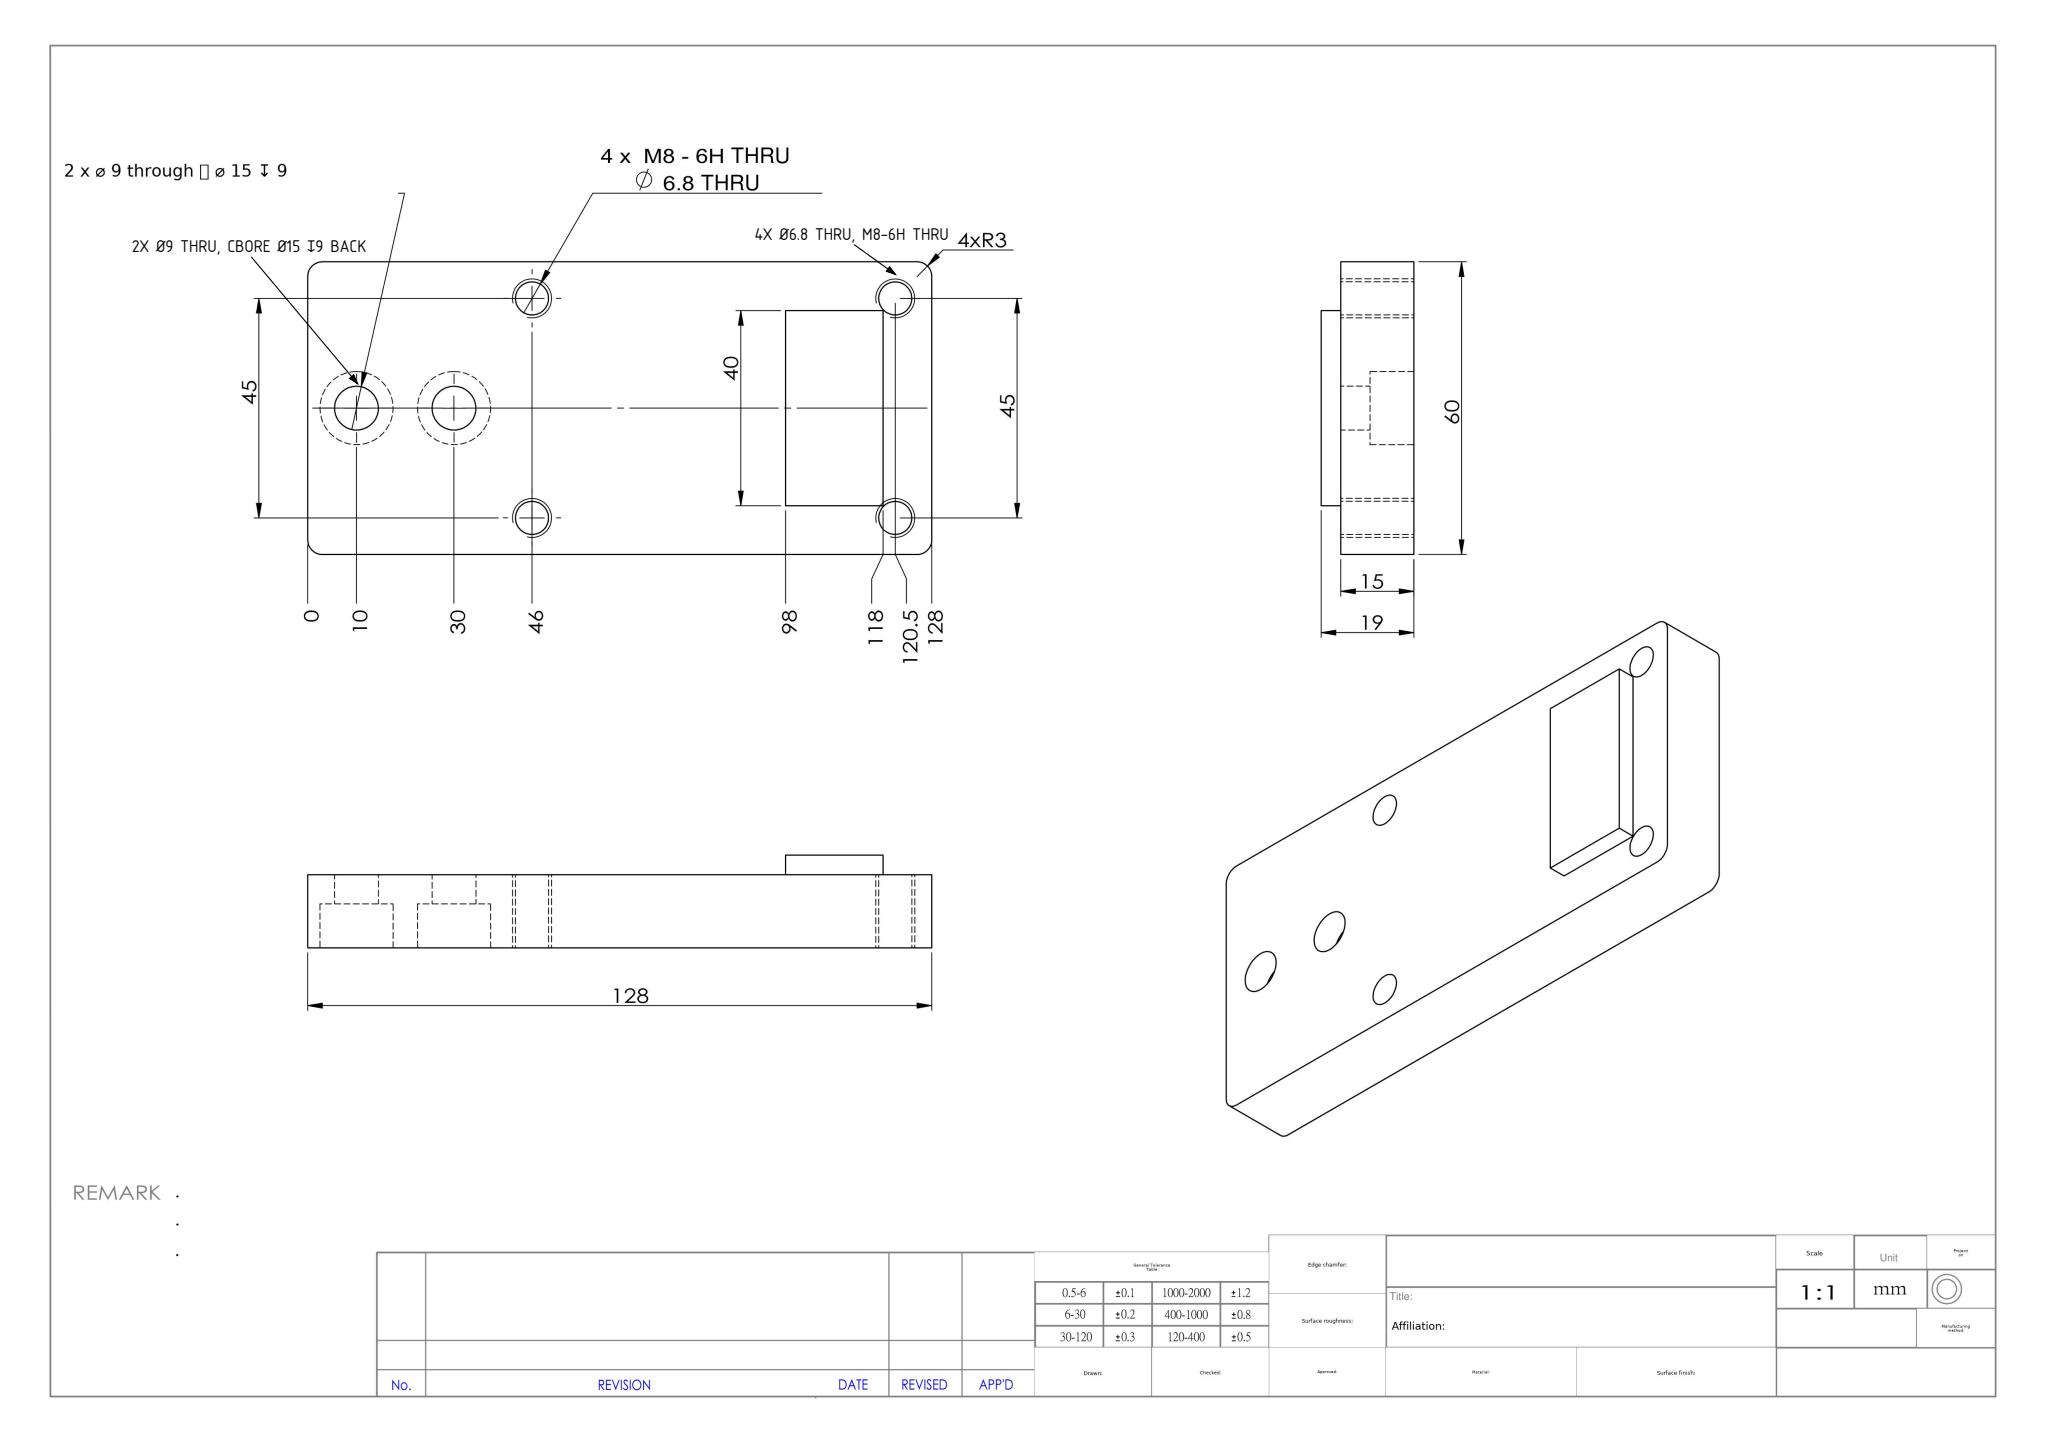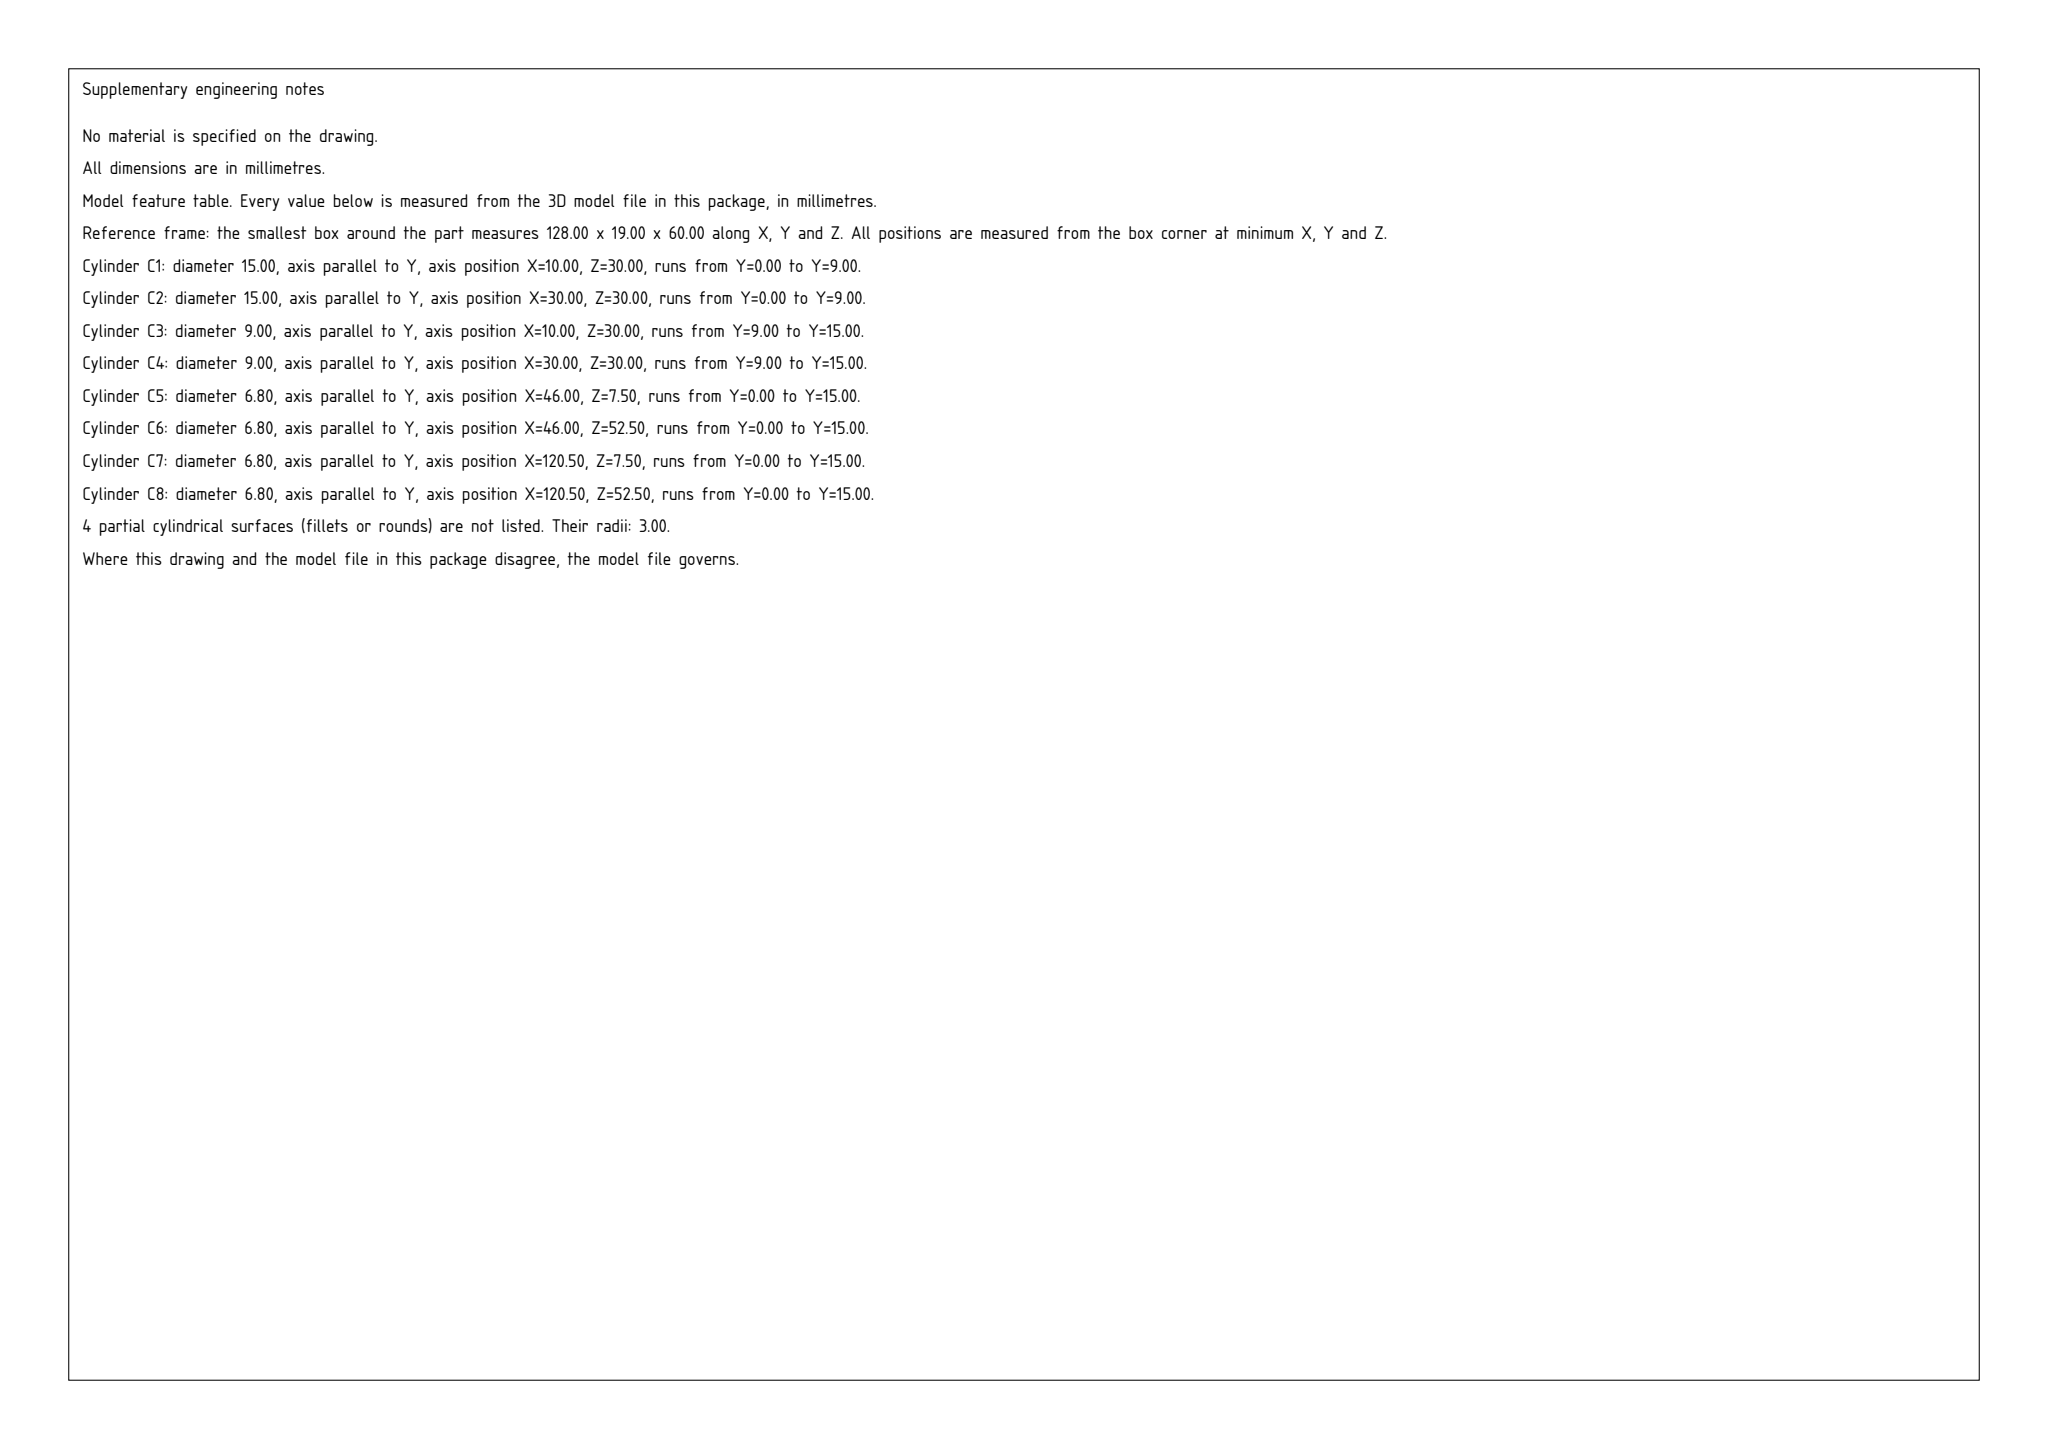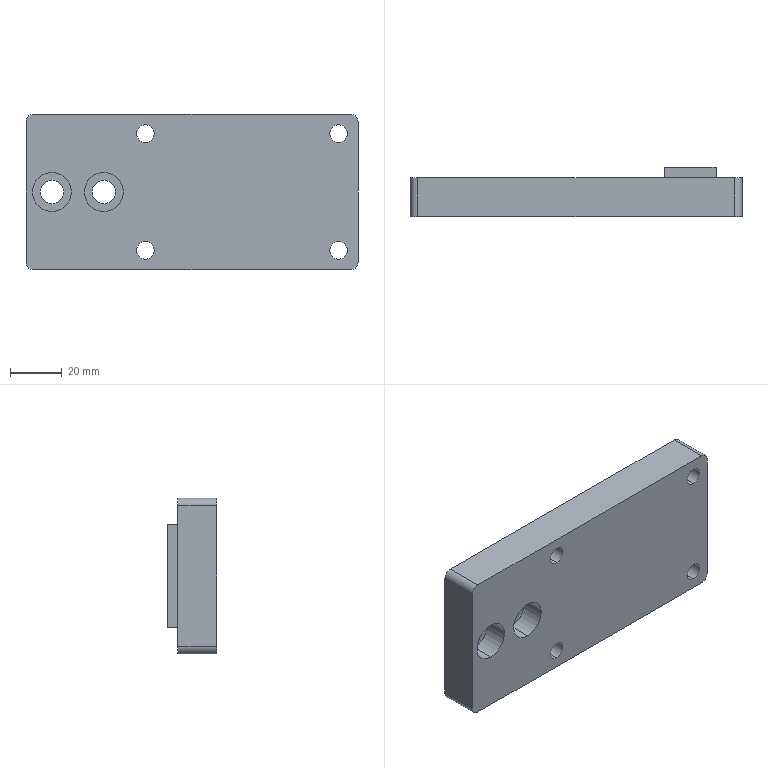Part | SolidWorks | mm | 1 solid | 33 faces | box 128 x 19 x 60 mm | volume 112161 mm3 | cylinder 20 | plane 13 | commonest cylinder face diameters 6.8 x8 15 x4 9 x4 6 x4
Drawing notes:
2 X Ø9 THRU, C'BORE Ø15 DP 9 FROM BACK FACE | from the solid: Ø15 bore y=0 to 9 at x=10 & x=30, z=30; Ø9 bore y=9 to 15 same axes
4 X Ø6.8 THRU, TAP M8-6H THRU (Ø6.8 = TAP DRILL) | from the solid: 4 x Ø6.8 holes thru 15 thk at (46,7.5),(46,52.5),(120.5,7.5),(120.5,52.5)
build123d program:
from build123d import *

# Parameters (mm, degrees)
SKETCH1_W                                         = 128
SKETCH1_H                                         = 60
BOSS_EXTRUDE1_DEPTH                               = 15
SKETCH2_W                                         = 20
SKETCH2_H                                         = 40
BOSS_EXTRUDE2_DEPTH                               = 4
FILLET1_R                                         = 3
HOLE_SIZE_BASED_ON_TYPE_1_HEXAGON_SOC_D           = 9
HOLE_SIZE_BASED_ON_TYPE_1_HEXAGON_SOC_CBORE_D     = 15
HOLE_SIZE_BASED_ON_TYPE_1_HEXAGON_SOC_CBORE_DEPTH = 9
M8_TAPPED_HOLE2_D                                 = 6.8


with BuildPart() as part:
    # Sketch1 → Boss-Extrude1 (new body)
    with BuildSketch(Plane(origin=(0, 0, 0), x_dir=(1, 0, 0), z_dir=(0, 1, 0))):
        Rectangle(SKETCH1_W, SKETCH1_H)
    extrude(amount=BOSS_EXTRUDE1_DEPTH)

    # Sketch2 → Boss-Extrude2 (add)
    with BuildSketch(Plane(origin=(0, 15, 0), x_dir=(1, 0, 0), z_dir=(0, 1, 0))):
        with Locations((44, 0)):
            Rectangle(SKETCH2_W, SKETCH2_H)
    extrude(amount=BOSS_EXTRUDE2_DEPTH)

    # Fillet1
    fillet1_edges = [part.edges().sort_by_distance(p)[0] for p in [
        (64, 7.5, 30),
        (-64, 7.5, 30),
        (-64, 7.5, -30),
        (64, 7.5, -30),
    ]]
    fillet(fillet1_edges, radius=FILLET1_R)

    # Hole Size _ based on_ Type 1 Hexagon Soc (through all)
    with Locations(Plane(origin=(0, 0, 0), x_dir=(-1, 0, 0), z_dir=(0, -1, 0))):
        with Locations((54, 0), (34, 0)):
            CounterBoreHole(HOLE_SIZE_BASED_ON_TYPE_1_HEXAGON_SOC_D / 2, HOLE_SIZE_BASED_ON_TYPE_1_HEXAGON_SOC_CBORE_D / 2, HOLE_SIZE_BASED_ON_TYPE_1_HEXAGON_SOC_CBORE_DEPTH)

    # M8 Tapped Hole2 (through all)
    with Locations(Plane(origin=(0, 0, 0), x_dir=(-1, 0, 0), z_dir=(0, -1, 0))):
        with Locations((18, 22.5), (-56.5, 22.5), (-56.5, -22.5), (18, -22.5)):
            Hole(M8_TAPPED_HOLE2_D / 2)


solid = part.part